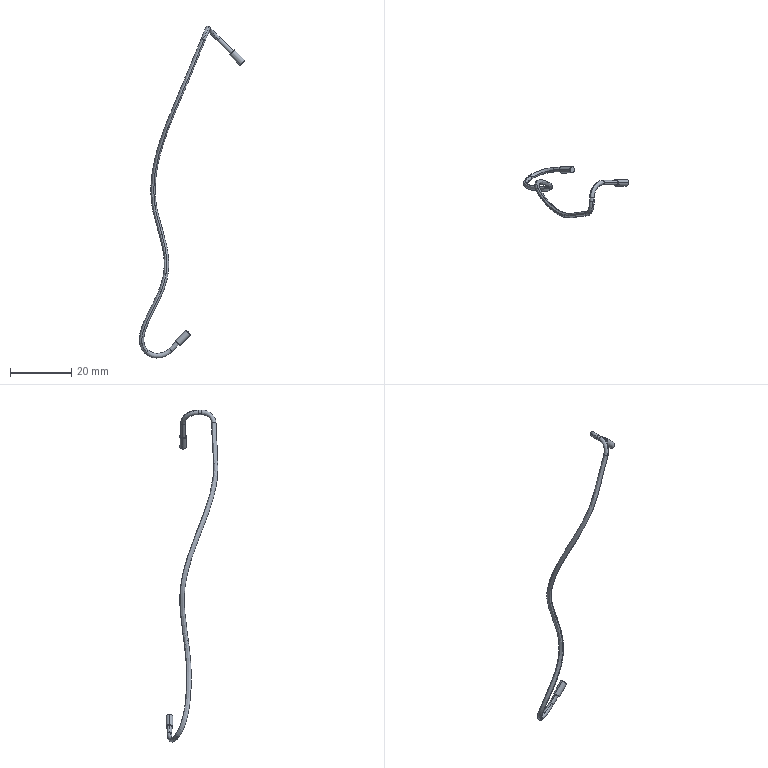Component | SolidWorks | Crijevo_paX-1 | 3 solids | 56 faces | box 34.33 x 16.92 x 108.11 mm | volume 98 mm3 | torus 20 | cylinder 20 | plane 8 | cone 4 | spline 4 | commonest cylinder face diameters 1.5 x10 1.3 x6 2.2 x4